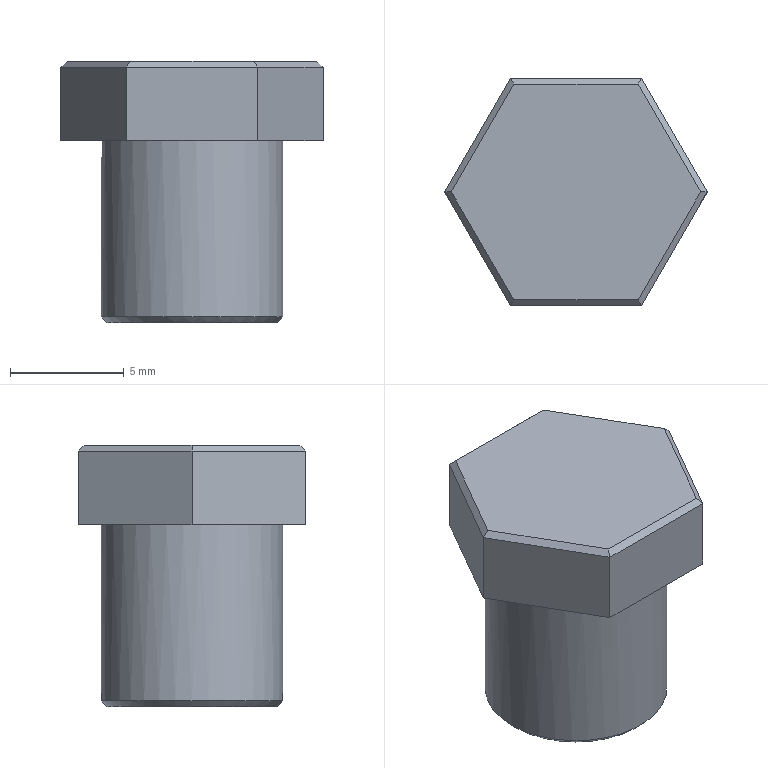Component | NX | BOLT_2 | 1 solid | 17 faces | box 11.55 x 10 x 11.5 mm | volume 703 mm3 | plane 15 | cylinder 1 | cone 1 | commonest cylinder face diameters 8 x1
STEP:
#1=CARTESIAN_POINT('',(0.,0.,0.));
#2=DIRECTION('',(0.,0.,1.));
#3=DIRECTION('',(1.,0.,0.));
#4=AXIS2_PLACEMENT_3D('',#1,#2,#3);
#5=CARTESIAN_POINT('',(-95.75,-10.75,52.));
#6=VERTEX_POINT('',#5);
#7=CARTESIAN_POINT('',(-92.,-10.75,52.));
#8=DIRECTION('',(0.,0.,-1.));
#9=DIRECTION('',(-1.,0.,0.));
#10=AXIS2_PLACEMENT_3D('',#7,#8,#9);
#11=CIRCLE('',#10,3.75);
#12=CARTESIAN_POINT('',(-92.,-10.75,52.));
#13=DIRECTION('',(0.,0.,-1.));
#14=DIRECTION('',(-1.,0.,0.));
#15=AXIS2_PLACEMENT_3D('',#12,#13,#14);
#16=PLANE('',#15);
#17=CARTESIAN_POINT('',(0.,0.));
#18=DIRECTION('',(1.,0.));
#19=AXIS2_PLACEMENT_2D('',#17,#18);
#20=CIRCLE('',#19,3.75);
#21=(GEOMETRIC_REPRESENTATION_CONTEXT(2)PARAMETRIC_REPRESENTATION_CONTEXT()REPRESENTATION_CONTEXT('',''));
#22=DEFINITIONAL_REPRESENTATION('',(#20),#21);
#23=PCURVE('',#16,#22);
#24=CARTESIAN_POINT('',(-92.,-10.75,52.25));
#25=DIRECTION('',(0.,0.,1.));
#26=DIRECTION('',(1.,0.,0.));
#27=AXIS2_PLACEMENT_3D('',#24,#25,#26);
#28=CONICAL_SURFACE('',#27,4.,0.7854);
#29=CARTESIAN_POINT('',(9.425,-0.25));
#30=DIRECTION('',(-1.,0.));
#31=VECTOR('',#30,1.);
#32=LINE('',#29,#31);
#33=(GEOMETRIC_REPRESENTATION_CONTEXT(2)PARAMETRIC_REPRESENTATION_CONTEXT()REPRESENTATION_CONTEXT('',''));
#34=DEFINITIONAL_REPRESENTATION('',(#32),#33);
#35=PCURVE('',#28,#34);
#36=SURFACE_CURVE('',#11,(#23,#35),.PCURVE_S1.);
#37=EDGE_CURVE('',#6,#6,#36,.T.);
#38=ORIENTED_EDGE('',*,*,#37,.T.);
#39=EDGE_LOOP('',(#38));
#40=FACE_BOUND('',#39,.T.);
#41=ADVANCED_FACE('',(#40),#16,.T.);
#42=CARTESIAN_POINT('',(-96.,-10.75,52.25));
#43=VERTEX_POINT('',#42);
#44=CARTESIAN_POINT('',(-88.,-10.75,52.25));
#45=VERTEX_POINT('',#44);
#46=CARTESIAN_POINT('',(-92.,-10.75,52.25));
#47=DIRECTION('',(0.,0.,1.));
#48=DIRECTION('',(-1.,0.,0.));
#49=AXIS2_PLACEMENT_3D('',#46,#47,#48);
#50=CIRCLE('',#49,4.);
#51=CARTESIAN_POINT('',(-92.,-10.75,52.));
#52=DIRECTION('',(0.,0.,1.));
#53=DIRECTION('',(1.,0.,0.));
#54=AXIS2_PLACEMENT_3D('',#51,#52,#53);
#55=CYLINDRICAL_SURFACE('',#54,4.);
#56=CARTESIAN_POINT('',(3.142,0.25));
#57=DIRECTION('',(1.,0.));
#58=VECTOR('',#57,1.);
#59=LINE('',#56,#58);
#60=(GEOMETRIC_REPRESENTATION_CONTEXT(2)PARAMETRIC_REPRESENTATION_CONTEXT()REPRESENTATION_CONTEXT('',''));
#61=DEFINITIONAL_REPRESENTATION('',(#59),#60);
#62=PCURVE('',#55,#61);
#63=CARTESIAN_POINT('',(3.142,0.));
#64=DIRECTION('',(1.,0.));
#65=VECTOR('',#64,1.);
#66=LINE('',#63,#65);
#67=(GEOMETRIC_REPRESENTATION_CONTEXT(2)PARAMETRIC_REPRESENTATION_CONTEXT()REPRESENTATION_CONTEXT('',''));
#68=DEFINITIONAL_REPRESENTATION('',(#66),#67);
#69=PCURVE('',#28,#68);
#70=SURFACE_CURVE('',#50,(#62,#69),.PCURVE_S1.);
#71=EDGE_CURVE('',#43,#45,#70,.T.);
#72=ORIENTED_EDGE('',*,*,#71,.T.);
#73=CARTESIAN_POINT('',(-88.,-10.75,60.));
#74=VERTEX_POINT('',#73);
#75=CARTESIAN_POINT('',(-88.,-10.75,52.25));
#76=CARTESIAN_POINT('',(-88.,-10.75,60.));
#77=B_SPLINE_CURVE_WITH_KNOTS('',1,(#75,#76),.UNSPECIFIED.,.F.,.F.,(2,2),(0.25,8.),.PIECEWISE_BEZIER_KNOTS.);
#78=CARTESIAN_POINT('',(6.283,0.));
#79=DIRECTION('',(0.,1.));
#80=VECTOR('',#79,1.);
#81=LINE('',#78,#80);
#82=(GEOMETRIC_REPRESENTATION_CONTEXT(2)PARAMETRIC_REPRESENTATION_CONTEXT()REPRESENTATION_CONTEXT('',''));
#83=DEFINITIONAL_REPRESENTATION('',(#81),#82);
#84=PCURVE('',#55,#83);
#85=CARTESIAN_POINT('',(0.,0.));
#86=DIRECTION('',(0.,1.));
#87=VECTOR('',#86,1.);
#88=LINE('',#85,#87);
#89=(GEOMETRIC_REPRESENTATION_CONTEXT(2)PARAMETRIC_REPRESENTATION_CONTEXT()REPRESENTATION_CONTEXT('',''));
#90=DEFINITIONAL_REPRESENTATION('',(#88),#89);
#91=PCURVE('',#55,#90);
#92=SEAM_CURVE('',#77,(#84,#91),.PCURVE_S1.);
#93=EDGE_CURVE('',#45,#74,#92,.T.);
#94=ORIENTED_EDGE('',*,*,#93,.T.);
#95=CARTESIAN_POINT('',(-92.,-10.75,60.));
#96=DIRECTION('',(0.,0.,-1.));
#97=DIRECTION('',(1.,0.,0.));
#98=AXIS2_PLACEMENT_3D('',#95,#96,#97);
#99=CIRCLE('',#98,4.);
#100=CARTESIAN_POINT('',(6.283,8.));
#101=DIRECTION('',(-1.,0.));
#102=VECTOR('',#101,1.);
#103=LINE('',#100,#102);
#104=(GEOMETRIC_REPRESENTATION_CONTEXT(2)PARAMETRIC_REPRESENTATION_CONTEXT()REPRESENTATION_CONTEXT('',''));
#105=DEFINITIONAL_REPRESENTATION('',(#103),#104);
#106=PCURVE('',#55,#105);
#107=CARTESIAN_POINT('',(-92.,-10.75,60.));
#108=DIRECTION('',(0.,0.,-1.));
#109=DIRECTION('',(-1.,0.,0.));
#110=AXIS2_PLACEMENT_3D('',#107,#108,#109);
#111=PLANE('',#110);
#112=CARTESIAN_POINT('',(0.,0.));
#113=DIRECTION('',(-1.,0.));
#114=AXIS2_PLACEMENT_2D('',#112,#113);
#115=CIRCLE('',#114,4.);
#116=(GEOMETRIC_REPRESENTATION_CONTEXT(2)PARAMETRIC_REPRESENTATION_CONTEXT()REPRESENTATION_CONTEXT('',''));
#117=DEFINITIONAL_REPRESENTATION('',(#115),#116);
#118=PCURVE('',#111,#117);
#119=SURFACE_CURVE('',#99,(#106,#118),.PCURVE_S1.);
#120=EDGE_CURVE('',#74,#74,#119,.T.);
#121=ORIENTED_EDGE('',*,*,#120,.T.);
#122=ORIENTED_EDGE('',*,*,#93,.F.);
#123=CARTESIAN_POINT('',(-92.,-10.75,52.25));
#124=DIRECTION('',(0.,0.,1.));
#125=DIRECTION('',(-1.,0.,0.));
#126=AXIS2_PLACEMENT_3D('',#123,#124,#125);
#127=CIRCLE('',#126,4.);
#128=CARTESIAN_POINT('',(-3.142,0.25));
#129=DIRECTION('',(1.,0.));
#130=VECTOR('',#129,1.);
#131=LINE('',#128,#130);
#132=(GEOMETRIC_REPRESENTATION_CONTEXT(2)PARAMETRIC_REPRESENTATION_CONTEXT()REPRESENTATION_CONTEXT('',''));
#133=DEFINITIONAL_REPRESENTATION('',(#131),#132);
#134=PCURVE('',#55,#133);
#135=CARTESIAN_POINT('',(3.142,0.));
#136=DIRECTION('',(1.,0.));
#137=VECTOR('',#136,1.);
#138=LINE('',#135,#137);
#139=(GEOMETRIC_REPRESENTATION_CONTEXT(2)PARAMETRIC_REPRESENTATION_CONTEXT()REPRESENTATION_CONTEXT('',''));
#140=DEFINITIONAL_REPRESENTATION('',(#138),#139);
#141=PCURVE('',#28,#140);
#142=SURFACE_CURVE('',#127,(#134,#141),.PCURVE_S1.);
#143=EDGE_CURVE('',#45,#43,#142,.T.);
#144=ORIENTED_EDGE('',*,*,#143,.T.);
#145=EDGE_LOOP('',(#72,#94,#121,#122,#144));
#146=FACE_BOUND('',#145,.T.);
#147=ADVANCED_FACE('',(#146),#55,.T.);
#148=CARTESIAN_POINT('',(-89.113,-5.75,63.25));
#149=VERTEX_POINT('',#148);
#150=CARTESIAN_POINT('',(-89.113,-5.75,60.));
#151=VERTEX_POINT('',#150);
#152=CARTESIAN_POINT('',(-89.113,-5.75,63.5));
#153=DIRECTION('',(0.,0.,-1.));
#154=VECTOR('',#153,1.);
#155=LINE('',#152,#154);
#156=CARTESIAN_POINT('',(-89.113,-5.75,63.5));
#157=DIRECTION('',(0.866,0.5,0.));
#158=DIRECTION('',(-0.5,0.866,0.));
#159=AXIS2_PLACEMENT_3D('',#156,#157,#158);
#160=PLANE('',#159);
#161=CARTESIAN_POINT('',(0.,0.));
#162=DIRECTION('',(0.,-1.));
#163=VECTOR('',#162,1.);
#164=LINE('',#161,#163);
#165=(GEOMETRIC_REPRESENTATION_CONTEXT(2)PARAMETRIC_REPRESENTATION_CONTEXT()REPRESENTATION_CONTEXT('',''));
#166=DEFINITIONAL_REPRESENTATION('',(#164),#165);
#167=PCURVE('',#160,#166);
#168=CARTESIAN_POINT('',(-94.887,-5.75,63.5));
#169=DIRECTION('',(0.,1.,0.));
#170=DIRECTION('',(-1.,0.,0.));
#171=AXIS2_PLACEMENT_3D('',#168,#169,#170);
#172=PLANE('',#171);
#173=CARTESIAN_POINT('',(-5.774,0.));
#174=DIRECTION('',(0.,-1.));
#175=VECTOR('',#174,1.);
#176=LINE('',#173,#175);
#177=(GEOMETRIC_REPRESENTATION_CONTEXT(2)PARAMETRIC_REPRESENTATION_CONTEXT()REPRESENTATION_CONTEXT('',''));
#178=DEFINITIONAL_REPRESENTATION('',(#176),#177);
#179=PCURVE('',#172,#178);
#180=SURFACE_CURVE('',#155,(#167,#179),.PCURVE_S1.);
#181=EDGE_CURVE('',#149,#151,#180,.T.);
#182=ORIENTED_EDGE('',*,*,#181,.F.);
#183=CARTESIAN_POINT('',(-86.226,-10.75,63.25));
#184=VERTEX_POINT('',#183);
#185=CARTESIAN_POINT('',(-86.226,-10.75,63.25));
#186=DIRECTION('',(0.5,-0.866,0.));
#187=VECTOR('',#186,1.);
#188=LINE('',#185,#187);
#189=CARTESIAN_POINT('',(-5.774,-0.25));
#190=DIRECTION('',(-1.,0.));
#191=VECTOR('',#190,1.);
#192=LINE('',#189,#191);
#193=(GEOMETRIC_REPRESENTATION_CONTEXT(2)PARAMETRIC_REPRESENTATION_CONTEXT()REPRESENTATION_CONTEXT('',''));
#194=DEFINITIONAL_REPRESENTATION('',(#192),#193);
#195=PCURVE('',#160,#194);
#196=CARTESIAN_POINT('',(-89.113,-5.75,63.25));
#197=DIRECTION('',(0.6124,0.3536,0.7071));
#198=DIRECTION('',(-0.5,0.866,-0.));
#199=AXIS2_PLACEMENT_3D('',#196,#197,#198);
#200=PLANE('',#199);
#201=CARTESIAN_POINT('',(-5.774,0.));
#202=DIRECTION('',(-1.,-0.));
#203=VECTOR('',#202,1.);
#204=LINE('',#201,#203);
#205=(GEOMETRIC_REPRESENTATION_CONTEXT(2)PARAMETRIC_REPRESENTATION_CONTEXT()REPRESENTATION_CONTEXT('',''));
#206=DEFINITIONAL_REPRESENTATION('',(#204),#205);
#207=PCURVE('',#200,#206);
#208=SURFACE_CURVE('',#188,(#195,#207),.PCURVE_S1.);
#209=EDGE_CURVE('',#149,#184,#208,.T.);
#210=ORIENTED_EDGE('',*,*,#209,.T.);
#211=CARTESIAN_POINT('',(-86.226,-10.75,60.));
#212=VERTEX_POINT('',#211);
#213=CARTESIAN_POINT('',(-86.226,-10.75,63.5));
#214=DIRECTION('',(0.,0.,-1.));
#215=VECTOR('',#214,1.);
#216=LINE('',#213,#215);
#217=CARTESIAN_POINT('',(-5.774,0.));
#218=DIRECTION('',(0.,-1.));
#219=VECTOR('',#218,1.);
#220=LINE('',#217,#219);
#221=(GEOMETRIC_REPRESENTATION_CONTEXT(2)PARAMETRIC_REPRESENTATION_CONTEXT()REPRESENTATION_CONTEXT('',''));
#222=DEFINITIONAL_REPRESENTATION('',(#220),#221);
#223=PCURVE('',#160,#222);
#224=CARTESIAN_POINT('',(-86.226,-10.75,63.5));
#225=DIRECTION('',(0.866,-0.5,0.));
#226=DIRECTION('',(0.5,0.866,0.));
#227=AXIS2_PLACEMENT_3D('',#224,#225,#226);
#228=PLANE('',#227);
#229=CARTESIAN_POINT('',(0.,0.));
#230=DIRECTION('',(0.,-1.));
#231=VECTOR('',#230,1.);
#232=LINE('',#229,#231);
#233=(GEOMETRIC_REPRESENTATION_CONTEXT(2)PARAMETRIC_REPRESENTATION_CONTEXT()REPRESENTATION_CONTEXT('',''));
#234=DEFINITIONAL_REPRESENTATION('',(#232),#233);
#235=PCURVE('',#228,#234);
#236=SURFACE_CURVE('',#216,(#223,#235),.PCURVE_S1.);
#237=EDGE_CURVE('',#184,#212,#236,.T.);
#238=ORIENTED_EDGE('',*,*,#237,.T.);
#239=CARTESIAN_POINT('',(-89.113,-5.75,60.));
#240=DIRECTION('',(0.5,-0.866,0.));
#241=VECTOR('',#240,1.);
#242=LINE('',#239,#241);
#243=CARTESIAN_POINT('',(0.,-3.5));
#244=DIRECTION('',(-1.,0.));
#245=VECTOR('',#244,1.);
#246=LINE('',#243,#245);
#247=(GEOMETRIC_REPRESENTATION_CONTEXT(2)PARAMETRIC_REPRESENTATION_CONTEXT()REPRESENTATION_CONTEXT('',''));
#248=DEFINITIONAL_REPRESENTATION('',(#246),#247);
#249=PCURVE('',#160,#248);
#250=CARTESIAN_POINT('',(-2.887,5.));
#251=DIRECTION('',(-0.5,-0.866));
#252=VECTOR('',#251,1.);
#253=LINE('',#250,#252);
#254=(GEOMETRIC_REPRESENTATION_CONTEXT(2)PARAMETRIC_REPRESENTATION_CONTEXT()REPRESENTATION_CONTEXT('',''));
#255=DEFINITIONAL_REPRESENTATION('',(#253),#254);
#256=PCURVE('',#111,#255);
#257=SURFACE_CURVE('',#242,(#249,#256),.PCURVE_S1.);
#258=EDGE_CURVE('',#151,#212,#257,.T.);
#259=ORIENTED_EDGE('',*,*,#258,.F.);
#260=EDGE_LOOP('',(#182,#210,#238,#259));
#261=FACE_BOUND('',#260,.T.);
#262=ADVANCED_FACE('',(#261),#160,.T.);
#263=ORIENTED_EDGE('',*,*,#237,.F.);
#264=CARTESIAN_POINT('',(-89.113,-15.75,63.25));
#265=VERTEX_POINT('',#264);
#266=CARTESIAN_POINT('',(-89.113,-15.75,63.25));
#267=DIRECTION('',(-0.5,-0.866,0.));
#268=VECTOR('',#267,1.);
#269=LINE('',#266,#268);
#270=CARTESIAN_POINT('',(-5.774,-0.25));
#271=DIRECTION('',(-1.,0.));
#272=VECTOR('',#271,1.);
#273=LINE('',#270,#272);
#274=(GEOMETRIC_REPRESENTATION_CONTEXT(2)PARAMETRIC_REPRESENTATION_CONTEXT()REPRESENTATION_CONTEXT('',''));
#275=DEFINITIONAL_REPRESENTATION('',(#273),#274);
#276=PCURVE('',#228,#275);
#277=CARTESIAN_POINT('',(-86.226,-10.75,63.25));
#278=DIRECTION('',(0.6124,-0.3536,0.7071));
#279=DIRECTION('',(0.5,0.866,-0.));
#280=AXIS2_PLACEMENT_3D('',#277,#278,#279);
#281=PLANE('',#280);
#282=CARTESIAN_POINT('',(-5.774,-0.));
#283=DIRECTION('',(-1.,0.));
#284=VECTOR('',#283,1.);
#285=LINE('',#282,#284);
#286=(GEOMETRIC_REPRESENTATION_CONTEXT(2)PARAMETRIC_REPRESENTATION_CONTEXT()REPRESENTATION_CONTEXT('',''));
#287=DEFINITIONAL_REPRESENTATION('',(#285),#286);
#288=PCURVE('',#281,#287);
#289=SURFACE_CURVE('',#269,(#276,#288),.PCURVE_S1.);
#290=EDGE_CURVE('',#184,#265,#289,.T.);
#291=ORIENTED_EDGE('',*,*,#290,.T.);
#292=CARTESIAN_POINT('',(-89.113,-15.75,60.));
#293=VERTEX_POINT('',#292);
#294=CARTESIAN_POINT('',(-89.113,-15.75,63.5));
#295=DIRECTION('',(0.,0.,-1.));
#296=VECTOR('',#295,1.);
#297=LINE('',#294,#296);
#298=CARTESIAN_POINT('',(-5.774,0.));
#299=DIRECTION('',(0.,-1.));
#300=VECTOR('',#299,1.);
#301=LINE('',#298,#300);
#302=(GEOMETRIC_REPRESENTATION_CONTEXT(2)PARAMETRIC_REPRESENTATION_CONTEXT()REPRESENTATION_CONTEXT('',''));
#303=DEFINITIONAL_REPRESENTATION('',(#301),#302);
#304=PCURVE('',#228,#303);
#305=CARTESIAN_POINT('',(-89.113,-15.75,63.5));
#306=DIRECTION('',(-0.,-1.,0.));
#307=DIRECTION('',(1.,-0.,0.));
#308=AXIS2_PLACEMENT_3D('',#305,#306,#307);
#309=PLANE('',#308);
#310=CARTESIAN_POINT('',(0.,0.));
#311=DIRECTION('',(0.,-1.));
#312=VECTOR('',#311,1.);
#313=LINE('',#310,#312);
#314=(GEOMETRIC_REPRESENTATION_CONTEXT(2)PARAMETRIC_REPRESENTATION_CONTEXT()REPRESENTATION_CONTEXT('',''));
#315=DEFINITIONAL_REPRESENTATION('',(#313),#314);
#316=PCURVE('',#309,#315);
#317=SURFACE_CURVE('',#297,(#304,#316),.PCURVE_S1.);
#318=EDGE_CURVE('',#265,#293,#317,.T.);
#319=ORIENTED_EDGE('',*,*,#318,.T.);
#320=CARTESIAN_POINT('',(-86.226,-10.75,60.));
#321=DIRECTION('',(-0.5,-0.866,0.));
#322=VECTOR('',#321,1.);
#323=LINE('',#320,#322);
#324=CARTESIAN_POINT('',(0.,-3.5));
#325=DIRECTION('',(-1.,0.));
#326=VECTOR('',#325,1.);
#327=LINE('',#324,#326);
#328=(GEOMETRIC_REPRESENTATION_CONTEXT(2)PARAMETRIC_REPRESENTATION_CONTEXT()REPRESENTATION_CONTEXT('',''));
#329=DEFINITIONAL_REPRESENTATION('',(#327),#328);
#330=PCURVE('',#228,#329);
#331=CARTESIAN_POINT('',(-5.774,0.));
#332=DIRECTION('',(0.5,-0.866));
#333=VECTOR('',#332,1.);
#334=LINE('',#331,#333);
#335=(GEOMETRIC_REPRESENTATION_CONTEXT(2)PARAMETRIC_REPRESENTATION_CONTEXT()REPRESENTATION_CONTEXT('',''));
#336=DEFINITIONAL_REPRESENTATION('',(#334),#335);
#337=PCURVE('',#111,#336);
#338=SURFACE_CURVE('',#323,(#330,#337),.PCURVE_S1.);
#339=EDGE_CURVE('',#212,#293,#338,.T.);
#340=ORIENTED_EDGE('',*,*,#339,.F.);
#341=EDGE_LOOP('',(#263,#291,#319,#340));
#342=FACE_BOUND('',#341,.T.);
#343=ADVANCED_FACE('',(#342),#228,.T.);
#344=ORIENTED_EDGE('',*,*,#318,.F.);
#345=CARTESIAN_POINT('',(-94.887,-15.75,63.25));
#346=VERTEX_POINT('',#345);
#347=CARTESIAN_POINT('',(-94.887,-15.75,63.25));
#348=DIRECTION('',(-1.,0.,0.));
#349=VECTOR('',#348,1.);
#350=LINE('',#347,#349);
#351=CARTESIAN_POINT('',(-5.774,-0.25));
#352=DIRECTION('',(-1.,0.));
#353=VECTOR('',#352,1.);
#354=LINE('',#351,#353);
#355=(GEOMETRIC_REPRESENTATION_CONTEXT(2)PARAMETRIC_REPRESENTATION_CONTEXT()REPRESENTATION_CONTEXT('',''));
#356=DEFINITIONAL_REPRESENTATION('',(#354),#355);
#357=PCURVE('',#309,#356);
#358=CARTESIAN_POINT('',(-89.113,-15.75,63.25));
#359=DIRECTION('',(-0.,-0.7071,0.7071));
#360=DIRECTION('',(1.,-0.,-0.));
#361=AXIS2_PLACEMENT_3D('',#358,#359,#360);
#362=PLANE('',#361);
#363=CARTESIAN_POINT('',(-5.774,-0.));
#364=DIRECTION('',(-1.,-0.));
#365=VECTOR('',#364,1.);
#366=LINE('',#363,#365);
#367=(GEOMETRIC_REPRESENTATION_CONTEXT(2)PARAMETRIC_REPRESENTATION_CONTEXT()REPRESENTATION_CONTEXT('',''));
#368=DEFINITIONAL_REPRESENTATION('',(#366),#367);
#369=PCURVE('',#362,#368);
#370=SURFACE_CURVE('',#350,(#357,#369),.PCURVE_S1.);
#371=EDGE_CURVE('',#265,#346,#370,.T.);
#372=ORIENTED_EDGE('',*,*,#371,.T.);
#373=CARTESIAN_POINT('',(-94.887,-15.75,60.));
#374=VERTEX_POINT('',#373);
#375=CARTESIAN_POINT('',(-94.887,-15.75,63.5));
#376=DIRECTION('',(0.,0.,-1.));
#377=VECTOR('',#376,1.);
#378=LINE('',#375,#377);
#379=CARTESIAN_POINT('',(-5.774,0.));
#380=DIRECTION('',(0.,-1.));
#381=VECTOR('',#380,1.);
#382=LINE('',#379,#381);
#383=(GEOMETRIC_REPRESENTATION_CONTEXT(2)PARAMETRIC_REPRESENTATION_CONTEXT()REPRESENTATION_CONTEXT('',''));
#384=DEFINITIONAL_REPRESENTATION('',(#382),#383);
#385=PCURVE('',#309,#384);
#386=CARTESIAN_POINT('',(-94.887,-15.75,63.5));
#387=DIRECTION('',(-0.866,-0.5,0.));
#388=DIRECTION('',(0.5,-0.866,0.));
#389=AXIS2_PLACEMENT_3D('',#386,#387,#388);
#390=PLANE('',#389);
#391=CARTESIAN_POINT('',(0.,0.));
#392=DIRECTION('',(0.,-1.));
#393=VECTOR('',#392,1.);
#394=LINE('',#391,#393);
#395=(GEOMETRIC_REPRESENTATION_CONTEXT(2)PARAMETRIC_REPRESENTATION_CONTEXT()REPRESENTATION_CONTEXT('',''));
#396=DEFINITIONAL_REPRESENTATION('',(#394),#395);
#397=PCURVE('',#390,#396);
#398=SURFACE_CURVE('',#378,(#385,#397),.PCURVE_S1.);
#399=EDGE_CURVE('',#346,#374,#398,.T.);
#400=ORIENTED_EDGE('',*,*,#399,.T.);
#401=CARTESIAN_POINT('',(-89.113,-15.75,60.));
#402=DIRECTION('',(-1.,0.,0.));
#403=VECTOR('',#402,1.);
#404=LINE('',#401,#403);
#405=CARTESIAN_POINT('',(0.,-3.5));
#406=DIRECTION('',(-1.,0.));
#407=VECTOR('',#406,1.);
#408=LINE('',#405,#407);
#409=(GEOMETRIC_REPRESENTATION_CONTEXT(2)PARAMETRIC_REPRESENTATION_CONTEXT()REPRESENTATION_CONTEXT('',''));
#410=DEFINITIONAL_REPRESENTATION('',(#408),#409);
#411=PCURVE('',#309,#410);
#412=CARTESIAN_POINT('',(-2.887,-5.));
#413=DIRECTION('',(1.,0.));
#414=VECTOR('',#413,1.);
#415=LINE('',#412,#414);
#416=(GEOMETRIC_REPRESENTATION_CONTEXT(2)PARAMETRIC_REPRESENTATION_CONTEXT()REPRESENTATION_CONTEXT('',''));
#417=DEFINITIONAL_REPRESENTATION('',(#415),#416);
#418=PCURVE('',#111,#417);
#419=SURFACE_CURVE('',#404,(#411,#418),.PCURVE_S1.);
#420=EDGE_CURVE('',#293,#374,#419,.T.);
#421=ORIENTED_EDGE('',*,*,#420,.F.);
#422=EDGE_LOOP('',(#344,#372,#400,#421));
#423=FACE_BOUND('',#422,.T.);
#424=ADVANCED_FACE('',(#423),#309,.T.);
#425=ORIENTED_EDGE('',*,*,#399,.F.);
#426=CARTESIAN_POINT('',(-97.774,-10.75,63.25));
#427=VERTEX_POINT('',#426);
#428=CARTESIAN_POINT('',(-97.774,-10.75,63.25));
#429=DIRECTION('',(-0.5,0.866,0.));
#430=VECTOR('',#429,1.);
#431=LINE('',#428,#430);
#432=CARTESIAN_POINT('',(-5.774,-0.25));
#433=DIRECTION('',(-1.,0.));
#434=VECTOR('',#433,1.);
#435=LINE('',#432,#434);
#436=(GEOMETRIC_REPRESENTATION_CONTEXT(2)PARAMETRIC_REPRESENTATION_CONTEXT()REPRESENTATION_CONTEXT('',''));
#437=DEFINITIONAL_REPRESENTATION('',(#435),#436);
#438=PCURVE('',#390,#437);
#439=CARTESIAN_POINT('',(-94.887,-15.75,63.25));
#440=DIRECTION('',(-0.6124,-0.3536,0.7071));
#441=DIRECTION('',(0.5,-0.866,0.));
#442=AXIS2_PLACEMENT_3D('',#439,#440,#441);
#443=PLANE('',#442);
#444=CARTESIAN_POINT('',(-5.774,0.));
#445=DIRECTION('',(-1.,0.));
#446=VECTOR('',#445,1.);
#447=LINE('',#444,#446);
#448=(GEOMETRIC_REPRESENTATION_CONTEXT(2)PARAMETRIC_REPRESENTATION_CONTEXT()REPRESENTATION_CONTEXT('',''));
#449=DEFINITIONAL_REPRESENTATION('',(#447),#448);
#450=PCURVE('',#443,#449);
#451=SURFACE_CURVE('',#431,(#438,#450),.PCURVE_S1.);
#452=EDGE_CURVE('',#346,#427,#451,.T.);
#453=ORIENTED_EDGE('',*,*,#452,.T.);
#454=CARTESIAN_POINT('',(-97.774,-10.75,60.));
#455=VERTEX_POINT('',#454);
#456=CARTESIAN_POINT('',(-97.774,-10.75,63.5));
#457=DIRECTION('',(0.,0.,-1.));
#458=VECTOR('',#457,1.);
#459=LINE('',#456,#458);
#460=CARTESIAN_POINT('',(-5.774,0.));
#461=DIRECTION('',(0.,-1.));
#462=VECTOR('',#461,1.);
#463=LINE('',#460,#462);
#464=(GEOMETRIC_REPRESENTATION_CONTEXT(2)PARAMETRIC_REPRESENTATION_CONTEXT()REPRESENTATION_CONTEXT('',''));
#465=DEFINITIONAL_REPRESENTATION('',(#463),#464);
#466=PCURVE('',#390,#465);
#467=CARTESIAN_POINT('',(-97.774,-10.75,63.5));
#468=DIRECTION('',(-0.866,0.5,0.));
#469=DIRECTION('',(-0.5,-0.866,0.));
#470=AXIS2_PLACEMENT_3D('',#467,#468,#469);
#471=PLANE('',#470);
#472=CARTESIAN_POINT('',(0.,0.));
#473=DIRECTION('',(0.,-1.));
#474=VECTOR('',#473,1.);
#475=LINE('',#472,#474);
#476=(GEOMETRIC_REPRESENTATION_CONTEXT(2)PARAMETRIC_REPRESENTATION_CONTEXT()REPRESENTATION_CONTEXT('',''));
#477=DEFINITIONAL_REPRESENTATION('',(#475),#476);
#478=PCURVE('',#471,#477);
#479=SURFACE_CURVE('',#459,(#466,#478),.PCURVE_S1.);
#480=EDGE_CURVE('',#427,#455,#479,.T.);
#481=ORIENTED_EDGE('',*,*,#480,.T.);
#482=CARTESIAN_POINT('',(-94.887,-15.75,60.));
#483=DIRECTION('',(-0.5,0.866,0.));
#484=VECTOR('',#483,1.);
#485=LINE('',#482,#484);
#486=CARTESIAN_POINT('',(0.,-3.5));
#487=DIRECTION('',(-1.,0.));
#488=VECTOR('',#487,1.);
#489=LINE('',#486,#488);
#490=(GEOMETRIC_REPRESENTATION_CONTEXT(2)PARAMETRIC_REPRESENTATION_CONTEXT()REPRESENTATION_CONTEXT('',''));
#491=DEFINITIONAL_REPRESENTATION('',(#489),#490);
#492=PCURVE('',#390,#491);
#493=CARTESIAN_POINT('',(2.887,-5.));
#494=DIRECTION('',(0.5,0.866));
#495=VECTOR('',#494,1.);
#496=LINE('',#493,#495);
#497=(GEOMETRIC_REPRESENTATION_CONTEXT(2)PARAMETRIC_REPRESENTATION_CONTEXT()REPRESENTATION_CONTEXT('',''));
#498=DEFINITIONAL_REPRESENTATION('',(#496),#497);
#499=PCURVE('',#111,#498);
#500=SURFACE_CURVE('',#485,(#492,#499),.PCURVE_S1.);
#501=EDGE_CURVE('',#374,#455,#500,.T.);
#502=ORIENTED_EDGE('',*,*,#501,.F.);
#503=EDGE_LOOP('',(#425,#453,#481,#502));
#504=FACE_BOUND('',#503,.T.);
#505=ADVANCED_FACE('',(#504),#390,.T.);
#506=ORIENTED_EDGE('',*,*,#480,.F.);
#507=CARTESIAN_POINT('',(-94.887,-5.75,63.25));
#508=VERTEX_POINT('',#507);
#509=CARTESIAN_POINT('',(-94.887,-5.75,63.25));
#510=DIRECTION('',(0.5,0.866,0.));
#511=VECTOR('',#510,1.);
#512=LINE('',#509,#511);
#513=CARTESIAN_POINT('',(-5.774,-0.25));
#514=DIRECTION('',(-1.,0.));
#515=VECTOR('',#514,1.);
#516=LINE('',#513,#515);
#517=(GEOMETRIC_REPRESENTATION_CONTEXT(2)PARAMETRIC_REPRESENTATION_CONTEXT()REPRESENTATION_CONTEXT('',''));
#518=DEFINITIONAL_REPRESENTATION('',(#516),#517);
#519=PCURVE('',#471,#518);
#520=CARTESIAN_POINT('',(-97.774,-10.75,63.25));
#521=DIRECTION('',(-0.6124,0.3536,0.7071));
#522=DIRECTION('',(-0.5,-0.866,-0.));
#523=AXIS2_PLACEMENT_3D('',#520,#521,#522);
#524=PLANE('',#523);
#525=CARTESIAN_POINT('',(-5.774,-0.));
#526=DIRECTION('',(-1.,0.));
#527=VECTOR('',#526,1.);
#528=LINE('',#525,#527);
#529=(GEOMETRIC_REPRESENTATION_CONTEXT(2)PARAMETRIC_REPRESENTATION_CONTEXT()REPRESENTATION_CONTEXT('',''));
#530=DEFINITIONAL_REPRESENTATION('',(#528),#529);
#531=PCURVE('',#524,#530);
#532=SURFACE_CURVE('',#512,(#519,#531),.PCURVE_S1.);
#533=EDGE_CURVE('',#427,#508,#532,.T.);
#534=ORIENTED_EDGE('',*,*,#533,.T.);
#535=CARTESIAN_POINT('',(-94.887,-5.75,60.));
#536=VERTEX_POINT('',#535);
#537=CARTESIAN_POINT('',(-94.887,-5.75,63.5));
#538=DIRECTION('',(0.,0.,-1.));
#539=VECTOR('',#538,1.);
#540=LINE('',#537,#539);
#541=CARTESIAN_POINT('',(-5.774,0.));
#542=DIRECTION('',(0.,-1.));
#543=VECTOR('',#542,1.);
#544=LINE('',#541,#543);
#545=(GEOMETRIC_REPRESENTATION_CONTEXT(2)PARAMETRIC_REPRESENTATION_CONTEXT()REPRESENTATION_CONTEXT('',''));
#546=DEFINITIONAL_REPRESENTATION('',(#544),#545);
#547=PCURVE('',#471,#546);
#548=CARTESIAN_POINT('',(0.,0.));
#549=DIRECTION('',(0.,-1.));
#550=VECTOR('',#549,1.);
#551=LINE('',#548,#550);
#552=(GEOMETRIC_REPRESENTATION_CONTEXT(2)PARAMETRIC_REPRESENTATION_CONTEXT()REPRESENTATION_CONTEXT('',''));
#553=DEFINITIONAL_REPRESENTATION('',(#551),#552);
#554=PCURVE('',#172,#553);
#555=SURFACE_CURVE('',#540,(#547,#554),.PCURVE_S1.);
#556=EDGE_CURVE('',#508,#536,#555,.T.);
#557=ORIENTED_EDGE('',*,*,#556,.T.);
#558=CARTESIAN_POINT('',(-97.774,-10.75,60.));
#559=DIRECTION('',(0.5,0.866,0.));
#560=VECTOR('',#559,1.);
#561=LINE('',#558,#560);
#562=CARTESIAN_POINT('',(0.,-3.5));
#563=DIRECTION('',(-1.,0.));
#564=VECTOR('',#563,1.);
#565=LINE('',#562,#564);
#566=(GEOMETRIC_REPRESENTATION_CONTEXT(2)PARAMETRIC_REPRESENTATION_CONTEXT()REPRESENTATION_CONTEXT('',''));
#567=DEFINITIONAL_REPRESENTATION('',(#565),#566);
#568=PCURVE('',#471,#567);
#569=CARTESIAN_POINT('',(5.774,0.));
#570=DIRECTION('',(-0.5,0.866));
#571=VECTOR('',#570,1.);
#572=LINE('',#569,#571);
#573=(GEOMETRIC_REPRESENTATION_CONTEXT(2)PARAMETRIC_REPRESENTATION_CONTEXT()REPRESENTATION_CONTEXT('',''));
#574=DEFINITIONAL_REPRESENTATION('',(#572),#573);
#575=PCURVE('',#111,#574);
#576=SURFACE_CURVE('',#561,(#568,#575),.PCURVE_S1.);
#577=EDGE_CURVE('',#455,#536,#576,.T.);
#578=ORIENTED_EDGE('',*,*,#577,.F.);
#579=EDGE_LOOP('',(#506,#534,#557,#578));
#580=FACE_BOUND('',#579,.T.);
#581=ADVANCED_FACE('',(#580),#471,.T.);
#582=ORIENTED_EDGE('',*,*,#556,.F.);
#583=CARTESIAN_POINT('',(-89.113,-5.75,63.25));
#584=DIRECTION('',(1.,-0.,0.));
#585=VECTOR('',#584,1.);
#586=LINE('',#583,#585);
#587=CARTESIAN_POINT('',(-5.774,-0.25));
#588=DIRECTION('',(-1.,0.));
#589=VECTOR('',#588,1.);
#590=LINE('',#587,#589);
#591=(GEOMETRIC_REPRESENTATION_CONTEXT(2)PARAMETRIC_REPRESENTATION_CONTEXT()REPRESENTATION_CONTEXT('',''));
#592=DEFINITIONAL_REPRESENTATION('',(#590),#591);
#593=PCURVE('',#172,#592);
#594=CARTESIAN_POINT('',(-94.887,-5.75,63.25));
#595=DIRECTION('',(0.,0.7071,0.7071));
#596=DIRECTION('',(-1.,0.,-0.));
#597=AXIS2_PLACEMENT_3D('',#594,#595,#596);
#598=PLANE('',#597);
#599=CARTESIAN_POINT('',(-5.774,0.));
#600=DIRECTION('',(-1.,-0.));
#601=VECTOR('',#600,1.);
#602=LINE('',#599,#601);
#603=(GEOMETRIC_REPRESENTATION_CONTEXT(2)PARAMETRIC_REPRESENTATION_CONTEXT()REPRESENTATION_CONTEXT('',''));
#604=DEFINITIONAL_REPRESENTATION('',(#602),#603);
#605=PCURVE('',#598,#604);
#606=SURFACE_CURVE('',#586,(#593,#605),.PCURVE_S1.);
#607=EDGE_CURVE('',#508,#149,#606,.T.);
#608=ORIENTED_EDGE('',*,*,#607,.T.);
#609=ORIENTED_EDGE('',*,*,#181,.T.);
#610=CARTESIAN_POINT('',(-94.887,-5.75,60.));
#611=DIRECTION('',(1.,-0.,0.));
#612=VECTOR('',#611,1.);
#613=LINE('',#610,#612);
#614=CARTESIAN_POINT('',(0.,-3.5));
#615=DIRECTION('',(-1.,0.));
#616=VECTOR('',#615,1.);
#617=LINE('',#614,#616);
#618=(GEOMETRIC_REPRESENTATION_CONTEXT(2)PARAMETRIC_REPRESENTATION_CONTEXT()REPRESENTATION_CONTEXT('',''));
#619=DEFINITIONAL_REPRESENTATION('',(#617),#618);
#620=PCURVE('',#172,#619);
#621=CARTESIAN_POINT('',(2.887,5.));
#622=DIRECTION('',(-1.,-0.));
#623=VECTOR('',#622,1.);
#624=LINE('',#621,#623);
#625=(GEOMETRIC_REPRESENTATION_CONTEXT(2)PARAMETRIC_REPRESENTATION_CONTEXT()REPRESENTATION_CONTEXT('',''));
#626=DEFINITIONAL_REPRESENTATION('',(#624),#625);
#627=PCURVE('',#111,#626);
#628=SURFACE_CURVE('',#613,(#620,#627),.PCURVE_S1.);
#629=EDGE_CURVE('',#536,#151,#628,.T.);
#630=ORIENTED_EDGE('',*,*,#629,.F.);
#631=EDGE_LOOP('',(#582,#608,#609,#630));
#632=FACE_BOUND('',#631,.T.);
#633=ADVANCED_FACE('',(#632),#172,.T.);
#634=CARTESIAN_POINT('',(-89.258,-15.5,63.5));
#635=VERTEX_POINT('',#634);
#636=CARTESIAN_POINT('',(-86.515,-10.75,63.5));
#637=VERTEX_POINT('',#636);
#638=CARTESIAN_POINT('',(-86.443,-10.625,63.5));
#639=DIRECTION('',(0.5,0.866,0.));
#640=VECTOR('',#639,1.);
#641=LINE('',#638,#640);
#642=CARTESIAN_POINT('',(-92.,-10.75,63.5));
#643=DIRECTION('',(0.,0.,-1.));
#644=DIRECTION('',(-1.,0.,0.));
#645=AXIS2_PLACEMENT_3D('',#642,#643,#644);
#646=PLANE('',#645);
#647=CARTESIAN_POINT('',(-5.557,0.125));
#648=DIRECTION('',(-0.5,0.866));
#649=VECTOR('',#648,1.);
#650=LINE('',#647,#649);
#651=(GEOMETRIC_REPRESENTATION_CONTEXT(2)PARAMETRIC_REPRESENTATION_CONTEXT()REPRESENTATION_CONTEXT('',''));
#652=DEFINITIONAL_REPRESENTATION('',(#650),#651);
#653=PCURVE('',#646,#652);
#654=CARTESIAN_POINT('',(0.,0.3536));
#655=DIRECTION('',(1.,-0.));
#656=VECTOR('',#655,1.);
#657=LINE('',#654,#656);
#658=(GEOMETRIC_REPRESENTATION_CONTEXT(2)PARAMETRIC_REPRESENTATION_CONTEXT()REPRESENTATION_CONTEXT('',''));
#659=DEFINITIONAL_REPRESENTATION('',(#657),#658);
#660=PCURVE('',#281,#659);
#661=SURFACE_CURVE('',#641,(#653,#660),.PCURVE_S1.);
#662=EDGE_CURVE('',#635,#637,#661,.T.);
#663=ORIENTED_EDGE('',*,*,#662,.T.);
#664=CARTESIAN_POINT('',(-89.258,-6.,63.5));
#665=VERTEX_POINT('',#664);
#666=CARTESIAN_POINT('',(-89.33,-5.875,63.5));
#667=DIRECTION('',(-0.5,0.866,0.));
#668=VECTOR('',#667,1.);
#669=LINE('',#666,#668);
#670=CARTESIAN_POINT('',(-2.67,4.875));
#671=DIRECTION('',(0.5,0.866));
#672=VECTOR('',#671,1.);
#673=LINE('',#670,#672);
#674=(GEOMETRIC_REPRESENTATION_CONTEXT(2)PARAMETRIC_REPRESENTATION_CONTEXT()REPRESENTATION_CONTEXT('',''));
#675=DEFINITIONAL_REPRESENTATION('',(#673),#674);
#676=PCURVE('',#646,#675);
#677=CARTESIAN_POINT('',(-0.,0.3536));
#678=DIRECTION('',(1.,0.));
#679=VECTOR('',#678,1.);
#680=LINE('',#677,#679);
#681=(GEOMETRIC_REPRESENTATION_CONTEXT(2)PARAMETRIC_REPRESENTATION_CONTEXT()REPRESENTATION_CONTEXT('',''));
#682=DEFINITIONAL_REPRESENTATION('',(#680),#681);
#683=PCURVE('',#200,#682);
#684=SURFACE_CURVE('',#669,(#676,#683),.PCURVE_S1.);
#685=EDGE_CURVE('',#637,#665,#684,.T.);
#686=ORIENTED_EDGE('',*,*,#685,.T.);
#687=CARTESIAN_POINT('',(-94.742,-6.,63.5));
#688=VERTEX_POINT('',#687);
#689=CARTESIAN_POINT('',(-94.887,-6.,63.5));
#690=DIRECTION('',(-1.,0.,0.));
#691=VECTOR('',#690,1.);
#692=LINE('',#689,#691);
#693=CARTESIAN_POINT('',(2.887,4.75));
#694=DIRECTION('',(1.,0.));
#695=VECTOR('',#694,1.);
#696=LINE('',#693,#695);
#697=(GEOMETRIC_REPRESENTATION_CONTEXT(2)PARAMETRIC_REPRESENTATION_CONTEXT()REPRESENTATION_CONTEXT('',''));
#698=DEFINITIONAL_REPRESENTATION('',(#696),#697);
#699=PCURVE('',#646,#698);
#700=CARTESIAN_POINT('',(-0.,0.3536));
#701=DIRECTION('',(1.,0.));
#702=VECTOR('',#701,1.);
#703=LINE('',#700,#702);
#704=(GEOMETRIC_REPRESENTATION_CONTEXT(2)PARAMETRIC_REPRESENTATION_CONTEXT()REPRESENTATION_CONTEXT('',''));
#705=DEFINITIONAL_REPRESENTATION('',(#703),#704);
#706=PCURVE('',#598,#705);
#707=SURFACE_CURVE('',#692,(#699,#706),.PCURVE_S1.);
#708=EDGE_CURVE('',#665,#688,#707,.T.);
#709=ORIENTED_EDGE('',*,*,#708,.T.);
#710=CARTESIAN_POINT('',(-97.485,-10.75,63.5));
#711=VERTEX_POINT('',#710);
#712=CARTESIAN_POINT('',(-97.557,-10.875,63.5));
#713=DIRECTION('',(-0.5,-0.866,0.));
#714=VECTOR('',#713,1.);
#715=LINE('',#712,#714);
#716=CARTESIAN_POINT('',(5.557,-0.125));
#717=DIRECTION('',(0.5,-0.866));
#718=VECTOR('',#717,1.);
#719=LINE('',#716,#718);
#720=(GEOMETRIC_REPRESENTATION_CONTEXT(2)PARAMETRIC_REPRESENTATION_CONTEXT()REPRESENTATION_CONTEXT('',''));
#721=DEFINITIONAL_REPRESENTATION('',(#719),#720);
#722=PCURVE('',#646,#721);
#723=CARTESIAN_POINT('',(0.,0.3536));
#724=DIRECTION('',(1.,-0.));
#725=VECTOR('',#724,1.);
#726=LINE('',#723,#725);
#727=(GEOMETRIC_REPRESENTATION_CONTEXT(2)PARAMETRIC_REPRESENTATION_CONTEXT()REPRESENTATION_CONTEXT('',''));
#728=DEFINITIONAL_REPRESENTATION('',(#726),#727);
#729=PCURVE('',#524,#728);
#730=SURFACE_CURVE('',#715,(#722,#729),.PCURVE_S1.);
#731=EDGE_CURVE('',#688,#711,#730,.T.);
#732=ORIENTED_EDGE('',*,*,#731,.T.);
#733=CARTESIAN_POINT('',(-94.742,-15.5,63.5));
#734=VERTEX_POINT('',#733);
#735=CARTESIAN_POINT('',(-94.67,-15.625,63.5));
#736=DIRECTION('',(0.5,-0.866,0.));
#737=VECTOR('',#736,1.);
#738=LINE('',#735,#737);
#739=CARTESIAN_POINT('',(2.67,-4.875));
#740=DIRECTION('',(-0.5,-0.866));
#741=VECTOR('',#740,1.);
#742=LINE('',#739,#741);
#743=(GEOMETRIC_REPRESENTATION_CONTEXT(2)PARAMETRIC_REPRESENTATION_CONTEXT()REPRESENTATION_CONTEXT('',''));
#744=DEFINITIONAL_REPRESENTATION('',(#742),#743);
#745=PCURVE('',#646,#744);
#746=CARTESIAN_POINT('',(-0.,0.3536));
#747=DIRECTION('',(1.,-0.));
#748=VECTOR('',#747,1.);
#749=LINE('',#746,#748);
#750=(GEOMETRIC_REPRESENTATION_CONTEXT(2)PARAMETRIC_REPRESENTATION_CONTEXT()REPRESENTATION_CONTEXT('',''));
#751=DEFINITIONAL_REPRESENTATION('',(#749),#750);
#752=PCURVE('',#443,#751);
#753=SURFACE_CURVE('',#738,(#745,#752),.PCURVE_S1.);
#754=EDGE_CURVE('',#711,#734,#753,.T.);
#755=ORIENTED_EDGE('',*,*,#754,.T.);
#756=CARTESIAN_POINT('',(-89.113,-15.5,63.5));
#757=DIRECTION('',(1.,-0.,0.));
#758=VECTOR('',#757,1.);
#759=LINE('',#756,#758);
#760=CARTESIAN_POINT('',(-2.887,-4.75));
#761=DIRECTION('',(-1.,-0.));
#762=VECTOR('',#761,1.);
#763=LINE('',#760,#762);
#764=(GEOMETRIC_REPRESENTATION_CONTEXT(2)PARAMETRIC_REPRESENTATION_CONTEXT()REPRESENTATION_CONTEXT('',''));
#765=DEFINITIONAL_REPRESENTATION('',(#763),#764);
#766=PCURVE('',#646,#765);
#767=CARTESIAN_POINT('',(-0.,0.3536));
#768=DIRECTION('',(1.,0.));
#769=VECTOR('',#768,1.);
#770=LINE('',#767,#769);
#771=(GEOMETRIC_REPRESENTATION_CONTEXT(2)PARAMETRIC_REPRESENTATION_CONTEXT()REPRESENTATION_CONTEXT('',''));
#772=DEFINITIONAL_REPRESENTATION('',(#770),#771);
#773=PCURVE('',#362,#772);
#774=SURFACE_CURVE('',#759,(#766,#773),.PCURVE_S1.);
#775=EDGE_CURVE('',#734,#635,#774,.T.);
#776=ORIENTED_EDGE('',*,*,#775,.T.);
#777=EDGE_LOOP('',(#663,#686,#709,#732,#755,#776));
#778=FACE_BOUND('',#777,.T.);
#779=ADVANCED_FACE('',(#778),#646,.F.);
#780=ORIENTED_EDGE('',*,*,#120,.F.);
#781=EDGE_LOOP('',(#780));
#782=FACE_BOUND('',#781,.T.);
#783=ORIENTED_EDGE('',*,*,#258,.T.);
#784=ORIENTED_EDGE('',*,*,#339,.T.);
#785=ORIENTED_EDGE('',*,*,#420,.T.);
#786=ORIENTED_EDGE('',*,*,#501,.T.);
#787=ORIENTED_EDGE('',*,*,#577,.T.);
#788=ORIENTED_EDGE('',*,*,#629,.T.);
#789=EDGE_LOOP('',(#783,#784,#785,#786,#787,#788));
#790=FACE_BOUND('',#789,.T.);
#791=ADVANCED_FACE('',(#782,#790),#111,.T.);
#792=CARTESIAN_POINT('',(-94.062,-14.321,64.679));
#793=DIRECTION('',(-0.378,-0.6547,-0.6547));
#794=VECTOR('',#793,1.);
#795=LINE('',#792,#794);
#796=CARTESIAN_POINT('',(-0.8248,2.02));
#797=DIRECTION('',(0.378,-0.9258));
#798=VECTOR('',#797,1.);
#799=LINE('',#796,#798);
#800=(GEOMETRIC_REPRESENTATION_CONTEXT(2)PARAMETRIC_REPRESENTATION_CONTEXT()REPRESENTATION_CONTEXT('',''));
#801=DEFINITIONAL_REPRESENTATION('',(#799),#800);
#802=PCURVE('',#443,#801);
#803=CARTESIAN_POINT('',(-4.949,2.02));
#804=DIRECTION('',(-0.378,-0.9258));
#805=VECTOR('',#804,1.);
#806=LINE('',#803,#805);
#807=(GEOMETRIC_REPRESENTATION_CONTEXT(2)PARAMETRIC_REPRESENTATION_CONTEXT()REPRESENTATION_CONTEXT('',''));
#808=DEFINITIONAL_REPRESENTATION('',(#806),#807);
#809=PCURVE('',#362,#808);
#810=SURFACE_CURVE('',#795,(#802,#809),.PCURVE_S1.);
#811=EDGE_CURVE('',#734,#346,#810,.T.);
#812=ORIENTED_EDGE('',*,*,#811,.F.);
#813=ORIENTED_EDGE('',*,*,#754,.F.);
#814=CARTESIAN_POINT('',(-96.124,-10.75,64.679));
#815=DIRECTION('',(0.7559,-0.,0.6547));
#816=VECTOR('',#815,1.);
#817=LINE('',#814,#816);
#818=CARTESIAN_POINT('',(-4.949,2.02));
#819=DIRECTION('',(0.378,0.9258));
#820=VECTOR('',#819,1.);
#821=LINE('',#818,#820);
#822=(GEOMETRIC_REPRESENTATION_CONTEXT(2)PARAMETRIC_REPRESENTATION_CONTEXT()REPRESENTATION_CONTEXT('',''));
#823=DEFINITIONAL_REPRESENTATION('',(#821),#822);
#824=PCURVE('',#443,#823);
#825=CARTESIAN_POINT('',(-0.8248,2.02));
#826=DIRECTION('',(-0.378,0.9258));
#827=VECTOR('',#826,1.);
#828=LINE('',#825,#827);
#829=(GEOMETRIC_REPRESENTATION_CONTEXT(2)PARAMETRIC_REPRESENTATION_CONTEXT()REPRESENTATION_CONTEXT('',''));
#830=DEFINITIONAL_REPRESENTATION('',(#828),#829);
#831=PCURVE('',#524,#830);
#832=SURFACE_CURVE('',#817,(#824,#831),.PCURVE_S1.);
#833=EDGE_CURVE('',#427,#711,#832,.T.);
#834=ORIENTED_EDGE('',*,*,#833,.F.);
#835=ORIENTED_EDGE('',*,*,#452,.F.);
#836=EDGE_LOOP('',(#812,#813,#834,#835));
#837=FACE_BOUND('',#836,.T.);
#838=ADVANCED_FACE('',(#837),#443,.T.);
#839=ORIENTED_EDGE('',*,*,#833,.T.);
#840=ORIENTED_EDGE('',*,*,#731,.F.);
#841=CARTESIAN_POINT('',(-94.062,-7.179,64.679));
#842=DIRECTION('',(0.378,-0.6547,0.6547));
#843=VECTOR('',#842,1.);
#844=LINE('',#841,#843);
#845=CARTESIAN_POINT('',(-4.949,2.02));
#846=DIRECTION('',(0.378,0.9258));
#847=VECTOR('',#846,1.);
#848=LINE('',#845,#847);
#849=(GEOMETRIC_REPRESENTATION_CONTEXT(2)PARAMETRIC_REPRESENTATION_CONTEXT()REPRESENTATION_CONTEXT('',''));
#850=DEFINITIONAL_REPRESENTATION('',(#848),#849);
#851=PCURVE('',#524,#850);
#852=CARTESIAN_POINT('',(-0.8248,2.02));
#853=DIRECTION('',(-0.378,0.9258));
#854=VECTOR('',#853,1.);
#855=LINE('',#852,#854);
#856=(GEOMETRIC_REPRESENTATION_CONTEXT(2)PARAMETRIC_REPRESENTATION_CONTEXT()REPRESENTATION_CONTEXT('',''));
#857=DEFINITIONAL_REPRESENTATION('',(#855),#856);
#858=PCURVE('',#598,#857);
#859=SURFACE_CURVE('',#844,(#851,#858),.PCURVE_S1.);
#860=EDGE_CURVE('',#508,#688,#859,.T.);
#861=ORIENTED_EDGE('',*,*,#860,.F.);
#862=ORIENTED_EDGE('',*,*,#533,.F.);
#863=EDGE_LOOP('',(#839,#840,#861,#862));
#864=FACE_BOUND('',#863,.T.);
#865=ADVANCED_FACE('',(#864),#524,.T.);
#866=ORIENTED_EDGE('',*,*,#811,.T.);
#867=ORIENTED_EDGE('',*,*,#371,.F.);
#868=CARTESIAN_POINT('',(-89.938,-14.321,64.679));
#869=DIRECTION('',(0.378,-0.6547,-0.6547));
#870=VECTOR('',#869,1.);
#871=LINE('',#868,#870);
#872=CARTESIAN_POINT('',(-0.8248,2.02));
#873=DIRECTION('',(0.378,-0.9258));
#874=VECTOR('',#873,1.);
#875=LINE('',#872,#874);
#876=(GEOMETRIC_REPRESENTATION_CONTEXT(2)PARAMETRIC_REPRESENTATION_CONTEXT()REPRESENTATION_CONTEXT('',''));
#877=DEFINITIONAL_REPRESENTATION('',(#875),#876);
#878=PCURVE('',#362,#877);
#879=CARTESIAN_POINT('',(-4.949,2.02));
#880=DIRECTION('',(-0.378,-0.9258));
#881=VECTOR('',#880,1.);
#882=LINE('',#879,#881);
#883=(GEOMETRIC_REPRESENTATION_CONTEXT(2)PARAMETRIC_REPRESENTATION_CONTEXT()REPRESENTATION_CONTEXT('',''));
#884=DEFINITIONAL_REPRESENTATION('',(#882),#883);
#885=PCURVE('',#281,#884);
#886=SURFACE_CURVE('',#871,(#878,#885),.PCURVE_S1.);
#887=EDGE_CURVE('',#635,#265,#886,.T.);
#888=ORIENTED_EDGE('',*,*,#887,.F.);
#889=ORIENTED_EDGE('',*,*,#775,.F.);
#890=EDGE_LOOP('',(#866,#867,#888,#889));
#891=FACE_BOUND('',#890,.T.);
#892=ADVANCED_FACE('',(#891),#362,.T.);
#893=ORIENTED_EDGE('',*,*,#860,.T.);
#894=ORIENTED_EDGE('',*,*,#708,.F.);
#895=CARTESIAN_POINT('',(-89.938,-7.179,64.679));
#896=DIRECTION('',(-0.378,-0.6547,0.6547));
#897=VECTOR('',#896,1.);
#898=LINE('',#895,#897);
#899=CARTESIAN_POINT('',(-4.949,2.02));
#900=DIRECTION('',(0.378,0.9258));
#901=VECTOR('',#900,1.);
#902=LINE('',#899,#901);
#903=(GEOMETRIC_REPRESENTATION_CONTEXT(2)PARAMETRIC_REPRESENTATION_CONTEXT()REPRESENTATION_CONTEXT('',''));
#904=DEFINITIONAL_REPRESENTATION('',(#902),#903);
#905=PCURVE('',#598,#904);
#906=CARTESIAN_POINT('',(-0.8248,2.02));
#907=DIRECTION('',(-0.378,0.9258));
#908=VECTOR('',#907,1.);
#909=LINE('',#906,#908);
#910=(GEOMETRIC_REPRESENTATION_CONTEXT(2)PARAMETRIC_REPRESENTATION_CONTEXT()REPRESENTATION_CONTEXT('',''));
#911=DEFINITIONAL_REPRESENTATION('',(#909),#910);
#912=PCURVE('',#200,#911);
#913=SURFACE_CURVE('',#898,(#905,#912),.PCURVE_S1.);
#914=EDGE_CURVE('',#149,#665,#913,.T.);
#915=ORIENTED_EDGE('',*,*,#914,.F.);
#916=ORIENTED_EDGE('',*,*,#607,.F.);
#917=EDGE_LOOP('',(#893,#894,#915,#916));
#918=FACE_BOUND('',#917,.T.);
#919=ADVANCED_FACE('',(#918),#598,.T.);
#920=ORIENTED_EDGE('',*,*,#887,.T.);
#921=ORIENTED_EDGE('',*,*,#290,.F.);
#922=CARTESIAN_POINT('',(-86.226,-10.75,63.25));
#923=DIRECTION('',(0.7559,-0.,-0.6547));
#924=VECTOR('',#923,1.);
#925=LINE('',#922,#924);
#926=CARTESIAN_POINT('',(0.,0.));
#927=DIRECTION('',(0.378,-0.9258));
#928=VECTOR('',#927,1.);
#929=LINE('',#926,#928);
#930=(GEOMETRIC_REPRESENTATION_CONTEXT(2)PARAMETRIC_REPRESENTATION_CONTEXT()REPRESENTATION_CONTEXT('',''));
#931=DEFINITIONAL_REPRESENTATION('',(#929),#930);
#932=PCURVE('',#281,#931);
#933=CARTESIAN_POINT('',(-5.774,0.));
#934=DIRECTION('',(-0.378,-0.9258));
#935=VECTOR('',#934,1.);
#936=LINE('',#933,#935);
#937=(GEOMETRIC_REPRESENTATION_CONTEXT(2)PARAMETRIC_REPRESENTATION_CONTEXT()REPRESENTATION_CONTEXT('',''));
#938=DEFINITIONAL_REPRESENTATION('',(#936),#937);
#939=PCURVE('',#200,#938);
#940=SURFACE_CURVE('',#925,(#932,#939),.PCURVE_S1.);
#941=EDGE_CURVE('',#637,#184,#940,.T.);
#942=ORIENTED_EDGE('',*,*,#941,.F.);
#943=ORIENTED_EDGE('',*,*,#662,.F.);
#944=EDGE_LOOP('',(#920,#921,#942,#943));
#945=FACE_BOUND('',#944,.T.);
#946=ADVANCED_FACE('',(#945),#281,.T.);
#947=ORIENTED_EDGE('',*,*,#914,.T.);
#948=ORIENTED_EDGE('',*,*,#685,.F.);
#949=ORIENTED_EDGE('',*,*,#941,.T.);
#950=ORIENTED_EDGE('',*,*,#209,.F.);
#951=EDGE_LOOP('',(#947,#948,#949,#950));
#952=FACE_BOUND('',#951,.T.);
#953=ADVANCED_FACE('',(#952),#200,.T.);
#954=ORIENTED_EDGE('',*,*,#37,.F.);
#955=CARTESIAN_POINT('',(-95.75,-10.75,52.));
#956=CARTESIAN_POINT('',(-96.,-10.75,52.25));
#957=B_SPLINE_CURVE_WITH_KNOTS('',1,(#955,#956),.UNSPECIFIED.,.F.,.F.,(2,2),(-0.3536,0.),.PIECEWISE_BEZIER_KNOTS.);
#958=CARTESIAN_POINT('',(9.425,0.));
#959=DIRECTION('',(0.,1.));
#960=VECTOR('',#959,1.);
#961=LINE('',#958,#960);
#962=(GEOMETRIC_REPRESENTATION_CONTEXT(2)PARAMETRIC_REPRESENTATION_CONTEXT()REPRESENTATION_CONTEXT('',''));
#963=DEFINITIONAL_REPRESENTATION('',(#961),#962);
#964=PCURVE('',#28,#963);
#965=CARTESIAN_POINT('',(3.142,0.));
#966=DIRECTION('',(0.,1.));
#967=VECTOR('',#966,1.);
#968=LINE('',#965,#967);
#969=(GEOMETRIC_REPRESENTATION_CONTEXT(2)PARAMETRIC_REPRESENTATION_CONTEXT()REPRESENTATION_CONTEXT('',''));
#970=DEFINITIONAL_REPRESENTATION('',(#968),#969);
#971=PCURVE('',#28,#970);
#972=SEAM_CURVE('',#957,(#964,#971),.PCURVE_S1.);
#973=EDGE_CURVE('',#6,#43,#972,.T.);
#974=ORIENTED_EDGE('',*,*,#973,.T.);
#975=ORIENTED_EDGE('',*,*,#143,.F.);
#976=ORIENTED_EDGE('',*,*,#71,.F.);
#977=ORIENTED_EDGE('',*,*,#973,.F.);
#978=EDGE_LOOP('',(#954,#974,#975,#976,#977));
#979=FACE_BOUND('',#978,.T.);
#980=ADVANCED_FACE('',(#979),#28,.T.);
#981=CLOSED_SHELL('',(#41,#147,#262,#343,#424,#505,#581,#633,#779,#791,#838,#865,#892,#919,#946,#953,#980));
#982=MANIFOLD_SOLID_BREP('',#981);
#983=(LENGTH_UNIT()NAMED_UNIT(*)SI_UNIT(.MILLI.,.METRE.));
#984=UNCERTAINTY_MEASURE_WITH_UNIT(LENGTH_MEASURE(0.000001),#983,'','');
#985=(NAMED_UNIT(*)PLANE_ANGLE_UNIT()SI_UNIT($,.RADIAN.));
#986=(NAMED_UNIT(*)SI_UNIT($,.STERADIAN.)SOLID_ANGLE_UNIT());
#987=(GEOMETRIC_REPRESENTATION_CONTEXT(3)GLOBAL_UNCERTAINTY_ASSIGNED_CONTEXT((#984))GLOBAL_UNIT_ASSIGNED_CONTEXT((#983,#985,#986))REPRESENTATION_CONTEXT('',''));
#988=ADVANCED_BREP_SHAPE_REPRESENTATION('',(#4,#982),#987);